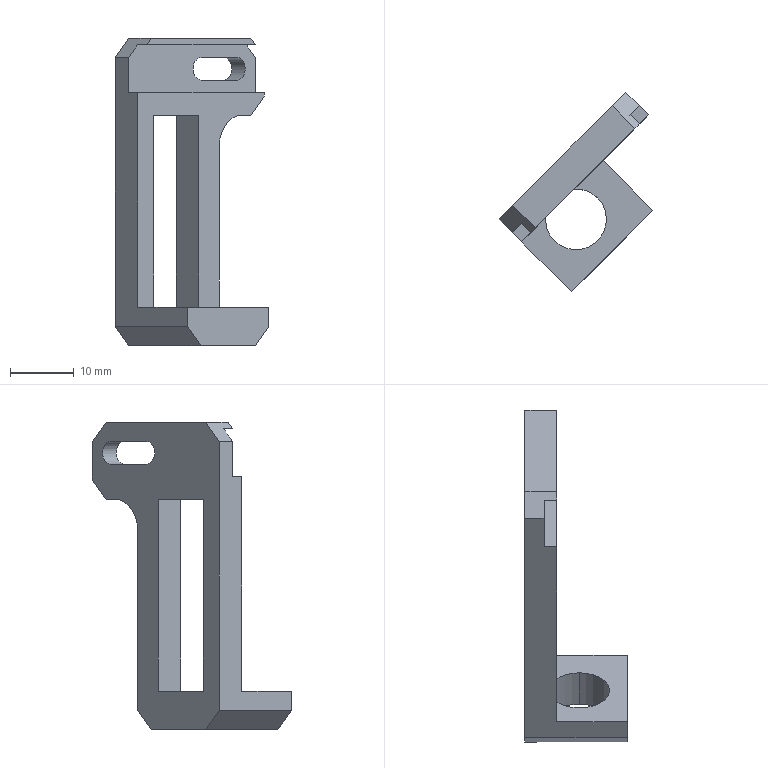Component | SolidWorks | InnerFineAdjustmentBlock-1 | 1 solid | 30 faces | box 24.04 x 31.11 x 48 mm | volume 3473 mm3 | plane 24 | cylinder 6 | commonest cylinder face diameters 3.5 x3 9.5 x2 10 x1
STEP:
#1=COLOUR_RGB('',0.7922,0.8196,0.9333);
#2=FILL_AREA_STYLE_COLOUR('',#1);
#3=FILL_AREA_STYLE('',(#2));
#4=SURFACE_STYLE_FILL_AREA(#3);
#5=SURFACE_SIDE_STYLE('',(#4));
#6=SURFACE_STYLE_USAGE(.BOTH.,#5);
#7=PRESENTATION_STYLE_ASSIGNMENT((#6));
#8=CARTESIAN_POINT('',(-6.312,5.308,0.5823));
#9=VERTEX_POINT('',#8);
#10=CARTESIAN_POINT('',(-6.263,5.357,0.6512));
#11=VERTEX_POINT('',#10);
#12=CARTESIAN_POINT('',(-6.263,5.357,0.5823));
#13=DIRECTION('',(-0.7071,0.7071,0.));
#14=DIRECTION('',(-0.7071,-0.7071,0.));
#15=AXIS2_PLACEMENT_3D('',#12,#13,#14);
#16=CIRCLE('',#15,0.0689);
#17=EDGE_CURVE('',#9,#11,#16,.T.);
#18=ORIENTED_EDGE('',*,*,#17,.F.);
#19=CARTESIAN_POINT('',(-6.395,5.391,0.5823));
#20=VERTEX_POINT('',#19);
#21=CARTESIAN_POINT('',(-5.95,4.946,0.5823));
#22=DIRECTION('',(-0.7071,0.7071,0.));
#23=VECTOR('',#22,39.37);
#24=LINE('',#21,#23);
#25=EDGE_CURVE('',#9,#20,#24,.T.);
#26=ORIENTED_EDGE('',*,*,#25,.T.);
#27=CARTESIAN_POINT('',(-6.347,5.44,0.6512));
#28=VERTEX_POINT('',#27);
#29=CARTESIAN_POINT('',(-6.347,5.44,0.5823));
#30=DIRECTION('',(-0.7071,0.7071,0.));
#31=DIRECTION('',(-0.7071,-0.7071,0.));
#32=AXIS2_PLACEMENT_3D('',#29,#30,#31);
#33=CIRCLE('',#32,0.0689);
#34=EDGE_CURVE('',#20,#28,#33,.T.);
#35=ORIENTED_EDGE('',*,*,#34,.T.);
#36=CARTESIAN_POINT('',(-5.901,4.995,0.6512));
#37=DIRECTION('',(0.7071,-0.7071,-0.));
#38=VECTOR('',#37,39.37);
#39=LINE('',#36,#38);
#40=EDGE_CURVE('',#28,#11,#39,.T.);
#41=ORIENTED_EDGE('',*,*,#40,.T.);
#42=EDGE_LOOP('',(#18,#26,#35,#41));
#43=FACE_OUTER_BOUND('',#42,.T.);
#44=CARTESIAN_POINT('',(-5.901,4.995,0.5823));
#45=DIRECTION('',(-0.7071,0.7071,0.));
#46=DIRECTION('',(-0.7071,-0.7071,0.));
#47=AXIS2_PLACEMENT_3D('',#44,#45,#46);
#48=CYLINDRICAL_SURFACE('',#47,0.0689);
#49=ADVANCED_FACE('',(#43),#48,.F.);
#50=CARTESIAN_POINT('',(-6.451,4.862,-0.8842));
#51=VERTEX_POINT('',#50);
#52=CARTESIAN_POINT('',(-6.187,5.127,-0.8842));
#53=VERTEX_POINT('',#52);
#54=CARTESIAN_POINT('',(-6.319,4.995,-0.8842));
#55=DIRECTION('',(0.,-0.,1.));
#56=DIRECTION('',(-0.7071,-0.7071,0.));
#57=AXIS2_PLACEMENT_3D('',#54,#55,#56);
#58=CIRCLE('',#57,0.187);
#59=EDGE_CURVE('',#51,#53,#58,.T.);
#60=ORIENTED_EDGE('',*,*,#59,.T.);
#61=CARTESIAN_POINT('',(-6.187,5.127,-1.12));
#62=VERTEX_POINT('',#61);
#63=CARTESIAN_POINT('',(-6.187,5.127,-0.7267));
#64=DIRECTION('',(-0.,0.,-1.));
#65=VECTOR('',#64,39.37);
#66=LINE('',#63,#65);
#67=EDGE_CURVE('',#53,#62,#66,.T.);
#68=ORIENTED_EDGE('',*,*,#67,.T.);
#69=CARTESIAN_POINT('',(-6.451,4.862,-1.12));
#70=VERTEX_POINT('',#69);
#71=CARTESIAN_POINT('',(-6.319,4.995,-1.12));
#72=DIRECTION('',(-0.,0.,-1.));
#73=DIRECTION('',(-0.7071,-0.7071,0.));
#74=AXIS2_PLACEMENT_3D('',#71,#72,#73);
#75=CIRCLE('',#74,0.187);
#76=EDGE_CURVE('',#62,#70,#75,.T.);
#77=ORIENTED_EDGE('',*,*,#76,.T.);
#78=CARTESIAN_POINT('',(-6.451,4.862,-0.7267));
#79=DIRECTION('',(-0.,0.,-1.));
#80=VECTOR('',#79,39.37);
#81=LINE('',#78,#80);
#82=EDGE_CURVE('',#51,#70,#81,.T.);
#83=ORIENTED_EDGE('',*,*,#82,.F.);
#84=EDGE_LOOP('',(#60,#68,#77,#83));
#85=FACE_OUTER_BOUND('',#84,.T.);
#86=CARTESIAN_POINT('',(-6.319,4.995,-0.7267));
#87=DIRECTION('',(-0.,0.,-1.));
#88=DIRECTION('',(-0.7071,-0.7071,0.));
#89=AXIS2_PLACEMENT_3D('',#86,#87,#88);
#90=CYLINDRICAL_SURFACE('',#89,0.187);
#91=ADVANCED_FACE('',(#85),#90,.F.);
#92=CARTESIAN_POINT('',(-6.375,5.412,-1.12));
#93=VERTEX_POINT('',#92);
#94=CARTESIAN_POINT('',(-6.291,5.496,-1.002));
#95=VERTEX_POINT('',#94);
#96=CARTESIAN_POINT('',(-6.375,5.412,-1.12));
#97=DIRECTION('',(0.5,0.5,0.7071));
#98=VECTOR('',#97,39.37);
#99=LINE('',#96,#98);
#100=EDGE_CURVE('',#93,#95,#99,.T.);
#101=ORIENTED_EDGE('',*,*,#100,.F.);
#102=CARTESIAN_POINT('',(-6.709,5.078,-1.12));
#103=VERTEX_POINT('',#102);
#104=CARTESIAN_POINT('',(-6.792,4.995,-1.12));
#105=DIRECTION('',(0.7071,0.7071,0.));
#106=VECTOR('',#105,39.37);
#107=LINE('',#104,#106);
#108=EDGE_CURVE('',#103,#93,#107,.T.);
#109=ORIENTED_EDGE('',*,*,#108,.F.);
#110=CARTESIAN_POINT('',(-6.792,4.995,-1.002));
#111=VERTEX_POINT('',#110);
#112=CARTESIAN_POINT('',(-6.792,4.995,-1.002));
#113=DIRECTION('',(0.5,0.5,-0.7071));
#114=VECTOR('',#113,39.37);
#115=LINE('',#112,#114);
#116=EDGE_CURVE('',#111,#103,#115,.T.);
#117=ORIENTED_EDGE('',*,*,#116,.F.);
#118=CARTESIAN_POINT('',(-6.792,4.995,0.6512));
#119=VERTEX_POINT('',#118);
#120=CARTESIAN_POINT('',(-6.792,4.995,-1.12));
#121=DIRECTION('',(-0.,0.,-1.));
#122=VECTOR('',#121,39.37);
#123=LINE('',#120,#122);
#124=EDGE_CURVE('',#119,#111,#123,.T.);
#125=ORIENTED_EDGE('',*,*,#124,.F.);
#126=CARTESIAN_POINT('',(-6.709,5.078,0.7693));
#127=VERTEX_POINT('',#126);
#128=CARTESIAN_POINT('',(-6.709,5.078,0.7693));
#129=DIRECTION('',(-0.5,-0.5,-0.7071));
#130=VECTOR('',#129,39.37);
#131=LINE('',#128,#130);
#132=EDGE_CURVE('',#127,#119,#131,.T.);
#133=ORIENTED_EDGE('',*,*,#132,.F.);
#134=CARTESIAN_POINT('',(-6.096,5.691,0.7693));
#135=VERTEX_POINT('',#134);
#136=CARTESIAN_POINT('',(-6.792,4.995,0.7693));
#137=DIRECTION('',(-0.7071,-0.7071,-0.));
#138=VECTOR('',#137,39.37);
#139=LINE('',#136,#138);
#140=EDGE_CURVE('',#135,#127,#139,.T.);
#141=ORIENTED_EDGE('',*,*,#140,.F.);
#142=CARTESIAN_POINT('',(-6.013,5.774,0.6512));
#143=VERTEX_POINT('',#142);
#144=CARTESIAN_POINT('',(-6.013,5.774,0.6512));
#145=DIRECTION('',(-0.5,-0.5,0.7071));
#146=VECTOR('',#145,39.37);
#147=LINE('',#144,#146);
#148=EDGE_CURVE('',#143,#135,#147,.T.);
#149=ORIENTED_EDGE('',*,*,#148,.F.);
#150=CARTESIAN_POINT('',(-6.013,5.774,0.415));
#151=VERTEX_POINT('',#150);
#152=CARTESIAN_POINT('',(-6.013,5.774,-1.12));
#153=DIRECTION('',(0.,-0.,1.));
#154=VECTOR('',#153,39.37);
#155=LINE('',#152,#154);
#156=EDGE_CURVE('',#151,#143,#155,.T.);
#157=ORIENTED_EDGE('',*,*,#156,.F.);
#158=CARTESIAN_POINT('',(-6.096,5.691,0.2969));
#159=VERTEX_POINT('',#158);
#160=CARTESIAN_POINT('',(-6.096,5.691,0.2969));
#161=DIRECTION('',(0.5,0.5,0.7071));
#162=VECTOR('',#161,39.37);
#163=LINE('',#160,#162);
#164=EDGE_CURVE('',#159,#151,#163,.T.);
#165=ORIENTED_EDGE('',*,*,#164,.F.);
#166=CARTESIAN_POINT('',(-6.152,5.635,0.2969));
#167=VERTEX_POINT('',#166);
#168=CARTESIAN_POINT('',(-6.792,4.995,0.2969));
#169=DIRECTION('',(0.7071,0.7071,0.));
#170=VECTOR('',#169,39.37);
#171=LINE('',#168,#170);
#172=EDGE_CURVE('',#167,#159,#171,.T.);
#173=ORIENTED_EDGE('',*,*,#172,.F.);
#174=CARTESIAN_POINT('',(-6.291,5.496,0.1));
#175=VERTEX_POINT('',#174);
#176=CARTESIAN_POINT('',(-6.152,5.635,0.1));
#177=DIRECTION('',(-0.7071,0.7071,0.));
#178=DIRECTION('',(0.7071,0.7071,0.));
#179=AXIS2_PLACEMENT_3D('',#176,#177,#178);
#180=CIRCLE('',#179,0.1969);
#181=EDGE_CURVE('',#175,#167,#180,.T.);
#182=ORIENTED_EDGE('',*,*,#181,.F.);
#183=CARTESIAN_POINT('',(-6.291,5.496,-1.12));
#184=DIRECTION('',(0.,-0.,1.));
#185=VECTOR('',#184,39.37);
#186=LINE('',#183,#185);
#187=EDGE_CURVE('',#95,#175,#186,.T.);
#188=ORIENTED_EDGE('',*,*,#187,.F.);
#189=EDGE_LOOP('',(#101,#109,#117,#125,#133,#141,#149,#157,#165,#173,#182,#188));
#190=FACE_OUTER_BOUND('',#189,.T.);
#191=CARTESIAN_POINT('',(-6.416,5.371,-0.8842));
#192=VERTEX_POINT('',#191);
#193=CARTESIAN_POINT('',(-6.695,5.092,-0.8842));
#194=VERTEX_POINT('',#193);
#195=CARTESIAN_POINT('',(-6.792,4.995,-0.8842));
#196=DIRECTION('',(-0.7071,-0.7071,-0.));
#197=VECTOR('',#196,39.37);
#198=LINE('',#195,#197);
#199=EDGE_CURVE('',#192,#194,#198,.T.);
#200=ORIENTED_EDGE('',*,*,#199,.F.);
#201=CARTESIAN_POINT('',(-6.416,5.371,0.2969));
#202=VERTEX_POINT('',#201);
#203=CARTESIAN_POINT('',(-6.416,5.371,-1.12));
#204=DIRECTION('',(-0.,0.,-1.));
#205=VECTOR('',#204,39.37);
#206=LINE('',#203,#205);
#207=EDGE_CURVE('',#202,#192,#206,.T.);
#208=ORIENTED_EDGE('',*,*,#207,.F.);
#209=CARTESIAN_POINT('',(-6.695,5.092,0.2969));
#210=VERTEX_POINT('',#209);
#211=CARTESIAN_POINT('',(-6.792,4.995,0.2969));
#212=DIRECTION('',(0.7071,0.7071,0.));
#213=VECTOR('',#212,39.37);
#214=LINE('',#211,#213);
#215=EDGE_CURVE('',#210,#202,#214,.T.);
#216=ORIENTED_EDGE('',*,*,#215,.F.);
#217=CARTESIAN_POINT('',(-6.695,5.092,-1.12));
#218=DIRECTION('',(0.,-0.,1.));
#219=VECTOR('',#218,39.37);
#220=LINE('',#217,#219);
#221=EDGE_CURVE('',#194,#210,#220,.T.);
#222=ORIENTED_EDGE('',*,*,#221,.F.);
#223=EDGE_LOOP('',(#200,#208,#216,#222));
#224=FACE_BOUND('',#223,.T.);
#225=CARTESIAN_POINT('',(-6.124,5.663,0.6512));
#226=VERTEX_POINT('',#225);
#227=CARTESIAN_POINT('',(-6.124,5.663,0.5134));
#228=VERTEX_POINT('',#227);
#229=CARTESIAN_POINT('',(-6.124,5.663,0.5823));
#230=DIRECTION('',(-0.7071,0.7071,0.));
#231=DIRECTION('',(-0.7071,-0.7071,0.));
#232=AXIS2_PLACEMENT_3D('',#229,#230,#231);
#233=CIRCLE('',#232,0.0689);
#234=EDGE_CURVE('',#226,#228,#233,.T.);
#235=ORIENTED_EDGE('',*,*,#234,.F.);
#236=CARTESIAN_POINT('',(-6.792,4.995,0.6512));
#237=DIRECTION('',(0.7071,0.7071,0.));
#238=VECTOR('',#237,39.37);
#239=LINE('',#236,#238);
#240=EDGE_CURVE('',#28,#226,#239,.T.);
#241=ORIENTED_EDGE('',*,*,#240,.F.);
#242=ORIENTED_EDGE('',*,*,#34,.F.);
#243=CARTESIAN_POINT('',(-6.347,5.44,0.5134));
#244=VERTEX_POINT('',#243);
#245=CARTESIAN_POINT('',(-6.347,5.44,0.5823));
#246=DIRECTION('',(-0.7071,0.7071,0.));
#247=DIRECTION('',(-0.7071,-0.7071,0.));
#248=AXIS2_PLACEMENT_3D('',#245,#246,#247);
#249=CIRCLE('',#248,0.0689);
#250=EDGE_CURVE('',#244,#20,#249,.T.);
#251=ORIENTED_EDGE('',*,*,#250,.F.);
#252=CARTESIAN_POINT('',(-6.792,4.995,0.5134));
#253=DIRECTION('',(-0.7071,-0.7071,-0.));
#254=VECTOR('',#253,39.37);
#255=LINE('',#252,#254);
#256=EDGE_CURVE('',#228,#244,#255,.T.);
#257=ORIENTED_EDGE('',*,*,#256,.F.);
#258=EDGE_LOOP('',(#235,#241,#242,#251,#257));
#259=FACE_BOUND('',#258,.T.);
#260=CARTESIAN_POINT('',(-6.792,4.995,-1.12));
#261=DIRECTION('',(0.7071,-0.7071,-0.));
#262=DIRECTION('',(0.7071,0.7071,0.));
#263=AXIS2_PLACEMENT_3D('',#260,#261,#262);
#264=PLANE('',#263);
#265=ADVANCED_FACE('',(#190,#224,#259),#264,.F.);
#266=CARTESIAN_POINT('',(-5.846,5.05,-1.002));
#267=VERTEX_POINT('',#266);
#268=CARTESIAN_POINT('',(-5.846,5.05,-1.002));
#269=DIRECTION('',(0.7071,-0.7071,-0.));
#270=VECTOR('',#269,39.37);
#271=LINE('',#268,#270);
#272=EDGE_CURVE('',#95,#267,#271,.T.);
#273=ORIENTED_EDGE('',*,*,#272,.F.);
#274=ORIENTED_EDGE('',*,*,#187,.T.);
#275=CARTESIAN_POINT('',(-6.152,5.357,0.1));
#276=VERTEX_POINT('',#275);
#277=CARTESIAN_POINT('',(-5.846,5.05,0.1));
#278=DIRECTION('',(-0.7071,0.7071,0.));
#279=VECTOR('',#278,39.37);
#280=LINE('',#277,#279);
#281=EDGE_CURVE('',#276,#175,#280,.T.);
#282=ORIENTED_EDGE('',*,*,#281,.F.);
#283=CARTESIAN_POINT('',(-6.152,5.357,-0.8842));
#284=VERTEX_POINT('',#283);
#285=CARTESIAN_POINT('',(-6.152,5.357,-1.12));
#286=DIRECTION('',(0.,-0.,1.));
#287=VECTOR('',#286,39.37);
#288=LINE('',#285,#287);
#289=EDGE_CURVE('',#284,#276,#288,.T.);
#290=ORIENTED_EDGE('',*,*,#289,.F.);
#291=CARTESIAN_POINT('',(-5.846,5.05,-0.8842));
#292=VERTEX_POINT('',#291);
#293=CARTESIAN_POINT('',(-5.846,5.05,-0.8842));
#294=DIRECTION('',(-0.7071,0.7071,0.));
#295=VECTOR('',#294,39.37);
#296=LINE('',#293,#295);
#297=EDGE_CURVE('',#292,#284,#296,.T.);
#298=ORIENTED_EDGE('',*,*,#297,.F.);
#299=CARTESIAN_POINT('',(-5.846,5.05,-1.12));
#300=DIRECTION('',(0.,-0.,1.));
#301=VECTOR('',#300,39.37);
#302=LINE('',#299,#301);
#303=EDGE_CURVE('',#267,#292,#302,.T.);
#304=ORIENTED_EDGE('',*,*,#303,.F.);
#305=EDGE_LOOP('',(#273,#274,#282,#290,#298,#304));
#306=FACE_OUTER_BOUND('',#305,.T.);
#307=CARTESIAN_POINT('',(-5.846,5.05,-1.12));
#308=DIRECTION('',(-0.7071,-0.7071,-0.));
#309=DIRECTION('',(0.,-0.,1.));
#310=AXIS2_PLACEMENT_3D('',#307,#308,#309);
#311=PLANE('',#310);
#312=ADVANCED_FACE('',(#306),#311,.F.);
#313=CARTESIAN_POINT('',(-5.929,4.967,-1.12));
#314=VERTEX_POINT('',#313);
#315=CARTESIAN_POINT('',(-5.929,4.967,-1.12));
#316=DIRECTION('',(0.7071,-0.7071,-0.));
#317=VECTOR('',#316,39.37);
#318=LINE('',#315,#317);
#319=EDGE_CURVE('',#93,#314,#318,.T.);
#320=ORIENTED_EDGE('',*,*,#319,.F.);
#321=ORIENTED_EDGE('',*,*,#100,.T.);
#322=ORIENTED_EDGE('',*,*,#272,.T.);
#323=CARTESIAN_POINT('',(-5.846,5.05,-1.002));
#324=DIRECTION('',(0.5,0.5,0.7071));
#325=VECTOR('',#324,39.37);
#326=LINE('',#323,#325);
#327=EDGE_CURVE('',#314,#267,#326,.T.);
#328=ORIENTED_EDGE('',*,*,#327,.F.);
#329=EDGE_LOOP('',(#320,#321,#322,#328));
#330=FACE_OUTER_BOUND('',#329,.T.);
#331=CARTESIAN_POINT('',(-5.846,5.05,-1.002));
#332=DIRECTION('',(-0.5,-0.5,0.7071));
#333=DIRECTION('',(0.5,0.5,0.7071));
#334=AXIS2_PLACEMENT_3D('',#331,#332,#333);
#335=PLANE('',#334);
#336=ADVANCED_FACE('',(#330),#335,.F.);
#337=ORIENTED_EDGE('',*,*,#319,.T.);
#338=CARTESIAN_POINT('',(-6.263,4.633,-1.12));
#339=VERTEX_POINT('',#338);
#340=CARTESIAN_POINT('',(-6.347,4.549,-1.12));
#341=DIRECTION('',(0.7071,0.7071,0.));
#342=VECTOR('',#341,39.37);
#343=LINE('',#340,#342);
#344=EDGE_CURVE('',#339,#314,#343,.T.);
#345=ORIENTED_EDGE('',*,*,#344,.F.);
#346=CARTESIAN_POINT('',(-6.709,5.078,-1.12));
#347=DIRECTION('',(0.7071,-0.7071,-0.));
#348=VECTOR('',#347,39.37);
#349=LINE('',#346,#348);
#350=EDGE_CURVE('',#103,#339,#349,.T.);
#351=ORIENTED_EDGE('',*,*,#350,.F.);
#352=ORIENTED_EDGE('',*,*,#108,.T.);
#353=EDGE_LOOP('',(#337,#345,#351,#352));
#354=FACE_OUTER_BOUND('',#353,.T.);
#355=CARTESIAN_POINT('',(-6.319,4.995,-1.12));
#356=DIRECTION('',(-0.,0.,-1.));
#357=DIRECTION('',(-0.7071,-0.7071,0.));
#358=AXIS2_PLACEMENT_3D('',#355,#356,#357);
#359=CIRCLE('',#358,0.187);
#360=EDGE_CURVE('',#70,#62,#359,.T.);
#361=ORIENTED_EDGE('',*,*,#360,.F.);
#362=ORIENTED_EDGE('',*,*,#76,.F.);
#363=EDGE_LOOP('',(#361,#362));
#364=FACE_BOUND('',#363,.T.);
#365=CARTESIAN_POINT('',(-6.792,4.995,-1.12));
#366=DIRECTION('',(0.,-0.,1.));
#367=DIRECTION('',(0.7071,0.7071,0.));
#368=AXIS2_PLACEMENT_3D('',#365,#366,#367);
#369=PLANE('',#368);
#370=ADVANCED_FACE('',(#354,#364),#369,.F.);
#371=ORIENTED_EDGE('',*,*,#350,.T.);
#372=CARTESIAN_POINT('',(-6.347,4.549,-1.002));
#373=VERTEX_POINT('',#372);
#374=CARTESIAN_POINT('',(-6.347,4.549,-1.002));
#375=DIRECTION('',(0.5,0.5,-0.7071));
#376=VECTOR('',#375,39.37);
#377=LINE('',#374,#376);
#378=EDGE_CURVE('',#373,#339,#377,.T.);
#379=ORIENTED_EDGE('',*,*,#378,.F.);
#380=CARTESIAN_POINT('',(-6.792,4.995,-1.002));
#381=DIRECTION('',(0.7071,-0.7071,-0.));
#382=VECTOR('',#381,39.37);
#383=LINE('',#380,#382);
#384=EDGE_CURVE('',#111,#373,#383,.T.);
#385=ORIENTED_EDGE('',*,*,#384,.F.);
#386=ORIENTED_EDGE('',*,*,#116,.T.);
#387=EDGE_LOOP('',(#371,#379,#385,#386));
#388=FACE_OUTER_BOUND('',#387,.T.);
#389=CARTESIAN_POINT('',(-6.792,4.995,-1.002));
#390=DIRECTION('',(0.5,0.5,0.7071));
#391=DIRECTION('',(0.5,0.5,-0.7071));
#392=AXIS2_PLACEMENT_3D('',#389,#390,#391);
#393=PLANE('',#392);
#394=ADVANCED_FACE('',(#388),#393,.F.);
#395=CARTESIAN_POINT('',(-6.709,4.911,0.6512));
#396=VERTEX_POINT('',#395);
#397=CARTESIAN_POINT('',(-6.792,4.995,0.6512));
#398=DIRECTION('',(0.7071,-0.7071,-0.));
#399=VECTOR('',#398,39.37);
#400=LINE('',#397,#399);
#401=EDGE_CURVE('',#119,#396,#400,.T.);
#402=ORIENTED_EDGE('',*,*,#401,.F.);
#403=ORIENTED_EDGE('',*,*,#124,.T.);
#404=ORIENTED_EDGE('',*,*,#384,.T.);
#405=CARTESIAN_POINT('',(-6.347,4.549,-0.8842));
#406=VERTEX_POINT('',#405);
#407=CARTESIAN_POINT('',(-6.347,4.549,-1.12));
#408=DIRECTION('',(-0.,0.,-1.));
#409=VECTOR('',#408,39.37);
#410=LINE('',#407,#409);
#411=EDGE_CURVE('',#406,#373,#410,.T.);
#412=ORIENTED_EDGE('',*,*,#411,.F.);
#413=CARTESIAN_POINT('',(-6.653,4.856,-0.8842));
#414=VERTEX_POINT('',#413);
#415=CARTESIAN_POINT('',(-6.792,4.995,-0.8842));
#416=DIRECTION('',(0.7071,-0.7071,-0.));
#417=VECTOR('',#416,39.37);
#418=LINE('',#415,#417);
#419=EDGE_CURVE('',#414,#406,#418,.T.);
#420=ORIENTED_EDGE('',*,*,#419,.F.);
#421=CARTESIAN_POINT('',(-6.653,4.856,0.4347));
#422=VERTEX_POINT('',#421);
#423=CARTESIAN_POINT('',(-6.653,4.856,-1.12));
#424=DIRECTION('',(-0.,0.,-1.));
#425=VECTOR('',#424,39.37);
#426=LINE('',#423,#425);
#427=EDGE_CURVE('',#422,#414,#426,.T.);
#428=ORIENTED_EDGE('',*,*,#427,.F.);
#429=CARTESIAN_POINT('',(-6.709,4.911,0.4347));
#430=VERTEX_POINT('',#429);
#431=CARTESIAN_POINT('',(-6.792,4.995,0.4347));
#432=DIRECTION('',(0.7071,-0.7071,-0.));
#433=VECTOR('',#432,39.37);
#434=LINE('',#431,#433);
#435=EDGE_CURVE('',#430,#422,#434,.T.);
#436=ORIENTED_EDGE('',*,*,#435,.F.);
#437=CARTESIAN_POINT('',(-6.709,4.911,-1.12));
#438=DIRECTION('',(-0.,0.,-1.));
#439=VECTOR('',#438,39.37);
#440=LINE('',#437,#439);
#441=EDGE_CURVE('',#396,#430,#440,.T.);
#442=ORIENTED_EDGE('',*,*,#441,.F.);
#443=EDGE_LOOP('',(#402,#403,#404,#412,#420,#428,#436,#442));
#444=FACE_OUTER_BOUND('',#443,.T.);
#445=CARTESIAN_POINT('',(-6.792,4.995,-1.12));
#446=DIRECTION('',(0.7071,0.7071,0.));
#447=DIRECTION('',(-0.,0.,-1.));
#448=AXIS2_PLACEMENT_3D('',#445,#446,#447);
#449=PLANE('',#448);
#450=ADVANCED_FACE('',(#444),#449,.F.);
#451=ORIENTED_EDGE('',*,*,#401,.T.);
#452=CARTESIAN_POINT('',(-6.653,4.967,0.73));
#453=VERTEX_POINT('',#452);
#454=CARTESIAN_POINT('',(-6.625,4.995,0.7693));
#455=DIRECTION('',(-0.5,-0.5,-0.7071));
#456=VECTOR('',#455,39.37);
#457=LINE('',#454,#456);
#458=EDGE_CURVE('',#453,#396,#457,.T.);
#459=ORIENTED_EDGE('',*,*,#458,.F.);
#460=CARTESIAN_POINT('',(-6.597,4.911,0.73));
#461=VERTEX_POINT('',#460);
#462=CARTESIAN_POINT('',(-6.736,5.05,0.73));
#463=DIRECTION('',(-0.7071,0.7071,0.));
#464=VECTOR('',#463,39.37);
#465=LINE('',#462,#464);
#466=EDGE_CURVE('',#461,#453,#465,.T.);
#467=ORIENTED_EDGE('',*,*,#466,.F.);
#468=CARTESIAN_POINT('',(-6.569,4.939,0.7693));
#469=VERTEX_POINT('',#468);
#470=CARTESIAN_POINT('',(-6.569,4.939,0.7693));
#471=DIRECTION('',(-0.5,-0.5,-0.7071));
#472=VECTOR('',#471,39.37);
#473=LINE('',#470,#472);
#474=EDGE_CURVE('',#469,#461,#473,.T.);
#475=ORIENTED_EDGE('',*,*,#474,.F.);
#476=CARTESIAN_POINT('',(-6.709,5.078,0.7693));
#477=DIRECTION('',(0.7071,-0.7071,-0.));
#478=VECTOR('',#477,39.37);
#479=LINE('',#476,#478);
#480=EDGE_CURVE('',#127,#469,#479,.T.);
#481=ORIENTED_EDGE('',*,*,#480,.F.);
#482=ORIENTED_EDGE('',*,*,#132,.T.);
#483=EDGE_LOOP('',(#451,#459,#467,#475,#481,#482));
#484=FACE_OUTER_BOUND('',#483,.T.);
#485=CARTESIAN_POINT('',(-6.709,5.078,0.7693));
#486=DIRECTION('',(0.5,0.5,-0.7071));
#487=DIRECTION('',(-0.5,-0.5,-0.7071));
#488=AXIS2_PLACEMENT_3D('',#485,#486,#487);
#489=PLANE('',#488);
#490=ADVANCED_FACE('',(#484),#489,.F.);
#491=CARTESIAN_POINT('',(-5.957,5.551,0.7693));
#492=VERTEX_POINT('',#491);
#493=CARTESIAN_POINT('',(-6.096,5.691,0.7693));
#494=DIRECTION('',(0.7071,-0.7071,-0.));
#495=VECTOR('',#494,39.37);
#496=LINE('',#493,#495);
#497=EDGE_CURVE('',#135,#492,#496,.T.);
#498=ORIENTED_EDGE('',*,*,#497,.F.);
#499=ORIENTED_EDGE('',*,*,#140,.T.);
#500=ORIENTED_EDGE('',*,*,#480,.T.);
#501=CARTESIAN_POINT('',(-6.653,4.856,0.7693));
#502=DIRECTION('',(-0.7071,-0.7071,-0.));
#503=VECTOR('',#502,39.37);
#504=LINE('',#501,#503);
#505=EDGE_CURVE('',#492,#469,#504,.T.);
#506=ORIENTED_EDGE('',*,*,#505,.F.);
#507=EDGE_LOOP('',(#498,#499,#500,#506));
#508=FACE_OUTER_BOUND('',#507,.T.);
#509=CARTESIAN_POINT('',(-6.792,4.995,0.7693));
#510=DIRECTION('',(-0.,0.,-1.));
#511=DIRECTION('',(-0.7071,-0.7071,-0.));
#512=AXIS2_PLACEMENT_3D('',#509,#510,#511);
#513=PLANE('',#512);
#514=ADVANCED_FACE('',(#508),#513,.F.);
#515=ORIENTED_EDGE('',*,*,#497,.T.);
#516=CARTESIAN_POINT('',(-5.929,5.579,0.73));
#517=VERTEX_POINT('',#516);
#518=CARTESIAN_POINT('',(-5.873,5.635,0.6512));
#519=DIRECTION('',(-0.5,-0.5,0.7071));
#520=VECTOR('',#519,39.37);
#521=LINE('',#518,#520);
#522=EDGE_CURVE('',#517,#492,#521,.T.);
#523=ORIENTED_EDGE('',*,*,#522,.F.);
#524=CARTESIAN_POINT('',(-5.985,5.635,0.73));
#525=VERTEX_POINT('',#524);
#526=CARTESIAN_POINT('',(-6.068,5.719,0.73));
#527=DIRECTION('',(0.7071,-0.7071,-0.));
#528=VECTOR('',#527,39.37);
#529=LINE('',#526,#528);
#530=EDGE_CURVE('',#525,#517,#529,.T.);
#531=ORIENTED_EDGE('',*,*,#530,.F.);
#532=CARTESIAN_POINT('',(-5.929,5.691,0.6512));
#533=VERTEX_POINT('',#532);
#534=CARTESIAN_POINT('',(-5.929,5.691,0.6512));
#535=DIRECTION('',(-0.5,-0.5,0.7071));
#536=VECTOR('',#535,39.37);
#537=LINE('',#534,#536);
#538=EDGE_CURVE('',#533,#525,#537,.T.);
#539=ORIENTED_EDGE('',*,*,#538,.F.);
#540=CARTESIAN_POINT('',(-6.013,5.774,0.6512));
#541=DIRECTION('',(0.7071,-0.7071,-0.));
#542=VECTOR('',#541,39.37);
#543=LINE('',#540,#542);
#544=EDGE_CURVE('',#143,#533,#543,.T.);
#545=ORIENTED_EDGE('',*,*,#544,.F.);
#546=ORIENTED_EDGE('',*,*,#148,.T.);
#547=EDGE_LOOP('',(#515,#523,#531,#539,#545,#546));
#548=FACE_OUTER_BOUND('',#547,.T.);
#549=CARTESIAN_POINT('',(-6.013,5.774,0.6512));
#550=DIRECTION('',(-0.5,-0.5,-0.7071));
#551=DIRECTION('',(-0.5,-0.5,0.7071));
#552=AXIS2_PLACEMENT_3D('',#549,#550,#551);
#553=PLANE('',#552);
#554=ADVANCED_FACE('',(#548),#553,.F.);
#555=CARTESIAN_POINT('',(-5.873,5.635,0.415));
#556=VERTEX_POINT('',#555);
#557=CARTESIAN_POINT('',(-6.013,5.774,0.415));
#558=DIRECTION('',(0.7071,-0.7071,-0.));
#559=VECTOR('',#558,39.37);
#560=LINE('',#557,#559);
#561=EDGE_CURVE('',#151,#556,#560,.T.);
#562=ORIENTED_EDGE('',*,*,#561,.F.);
#563=ORIENTED_EDGE('',*,*,#156,.T.);
#564=ORIENTED_EDGE('',*,*,#544,.T.);
#565=CARTESIAN_POINT('',(-5.929,5.691,0.4347));
#566=VERTEX_POINT('',#565);
#567=CARTESIAN_POINT('',(-5.929,5.691,-1.12));
#568=DIRECTION('',(0.,-0.,1.));
#569=VECTOR('',#568,39.37);
#570=LINE('',#567,#569);
#571=EDGE_CURVE('',#566,#533,#570,.T.);
#572=ORIENTED_EDGE('',*,*,#571,.F.);
#573=CARTESIAN_POINT('',(-5.873,5.635,0.4347));
#574=VERTEX_POINT('',#573);
#575=CARTESIAN_POINT('',(-6.013,5.774,0.4347));
#576=DIRECTION('',(-0.7071,0.7071,0.));
#577=VECTOR('',#576,39.37);
#578=LINE('',#575,#577);
#579=EDGE_CURVE('',#574,#566,#578,.T.);
#580=ORIENTED_EDGE('',*,*,#579,.F.);
#581=CARTESIAN_POINT('',(-5.873,5.635,-1.12));
#582=DIRECTION('',(0.,-0.,1.));
#583=VECTOR('',#582,39.37);
#584=LINE('',#581,#583);
#585=EDGE_CURVE('',#556,#574,#584,.T.);
#586=ORIENTED_EDGE('',*,*,#585,.F.);
#587=EDGE_LOOP('',(#562,#563,#564,#572,#580,#586));
#588=FACE_OUTER_BOUND('',#587,.T.);
#589=CARTESIAN_POINT('',(-6.013,5.774,-1.12));
#590=DIRECTION('',(-0.7071,-0.7071,-0.));
#591=DIRECTION('',(0.,-0.,1.));
#592=AXIS2_PLACEMENT_3D('',#589,#590,#591);
#593=PLANE('',#592);
#594=ADVANCED_FACE('',(#588),#593,.F.);
#595=CARTESIAN_POINT('',(-5.957,5.551,0.2969));
#596=VERTEX_POINT('',#595);
#597=CARTESIAN_POINT('',(-6.096,5.691,0.2969));
#598=DIRECTION('',(0.7071,-0.7071,-0.));
#599=VECTOR('',#598,39.37);
#600=LINE('',#597,#599);
#601=EDGE_CURVE('',#159,#596,#600,.T.);
#602=ORIENTED_EDGE('',*,*,#601,.F.);
#603=ORIENTED_EDGE('',*,*,#164,.T.);
#604=ORIENTED_EDGE('',*,*,#561,.T.);
#605=CARTESIAN_POINT('',(-5.873,5.635,0.415));
#606=DIRECTION('',(0.5,0.5,0.7071));
#607=VECTOR('',#606,39.37);
#608=LINE('',#605,#607);
#609=EDGE_CURVE('',#596,#556,#608,.T.);
#610=ORIENTED_EDGE('',*,*,#609,.F.);
#611=EDGE_LOOP('',(#602,#603,#604,#610));
#612=FACE_OUTER_BOUND('',#611,.T.);
#613=CARTESIAN_POINT('',(-6.013,5.774,0.415));
#614=DIRECTION('',(-0.5,-0.5,0.7071));
#615=DIRECTION('',(0.5,0.5,0.7071));
#616=AXIS2_PLACEMENT_3D('',#613,#614,#615);
#617=PLANE('',#616);
#618=ADVANCED_FACE('',(#612),#617,.F.);
#619=ORIENTED_EDGE('',*,*,#601,.T.);
#620=CARTESIAN_POINT('',(-6.013,5.496,0.2969));
#621=VERTEX_POINT('',#620);
#622=CARTESIAN_POINT('',(-5.873,5.635,0.2969));
#623=DIRECTION('',(0.7071,0.7071,0.));
#624=VECTOR('',#623,39.37);
#625=LINE('',#622,#624);
#626=EDGE_CURVE('',#621,#596,#625,.T.);
#627=ORIENTED_EDGE('',*,*,#626,.F.);
#628=CARTESIAN_POINT('',(-5.873,5.357,0.2969));
#629=DIRECTION('',(0.7071,-0.7071,-0.));
#630=VECTOR('',#629,39.37);
#631=LINE('',#628,#630);
#632=EDGE_CURVE('',#167,#621,#631,.T.);
#633=ORIENTED_EDGE('',*,*,#632,.F.);
#634=ORIENTED_EDGE('',*,*,#172,.T.);
#635=EDGE_LOOP('',(#619,#627,#633,#634));
#636=FACE_OUTER_BOUND('',#635,.T.);
#637=CARTESIAN_POINT('',(-5.734,5.496,0.2969));
#638=DIRECTION('',(0.,-0.,1.));
#639=DIRECTION('',(0.7071,0.7071,0.));
#640=AXIS2_PLACEMENT_3D('',#637,#638,#639);
#641=PLANE('',#640);
#642=ADVANCED_FACE('',(#636),#641,.F.);
#643=ORIENTED_EDGE('',*,*,#281,.T.);
#644=ORIENTED_EDGE('',*,*,#181,.T.);
#645=ORIENTED_EDGE('',*,*,#632,.T.);
#646=CARTESIAN_POINT('',(-6.013,5.496,0.1));
#647=DIRECTION('',(-0.7071,0.7071,0.));
#648=DIRECTION('',(0.7071,0.7071,0.));
#649=AXIS2_PLACEMENT_3D('',#646,#647,#648);
#650=CIRCLE('',#649,0.1969);
#651=EDGE_CURVE('',#276,#621,#650,.T.);
#652=ORIENTED_EDGE('',*,*,#651,.F.);
#653=EDGE_LOOP('',(#643,#644,#645,#652));
#654=FACE_OUTER_BOUND('',#653,.T.);
#655=CARTESIAN_POINT('',(-5.873,5.357,0.1));
#656=DIRECTION('',(0.7071,-0.7071,-0.));
#657=DIRECTION('',(0.7071,0.7071,0.));
#658=AXIS2_PLACEMENT_3D('',#655,#656,#657);
#659=CYLINDRICAL_SURFACE('',#658,0.1969);
#660=ADVANCED_FACE('',(#654),#659,.F.);
#661=CARTESIAN_POINT('',(-6.555,4.953,-0.8842));
#662=VERTEX_POINT('',#661);
#663=CARTESIAN_POINT('',(-6.249,4.647,-0.8842));
#664=DIRECTION('',(0.7071,-0.7071,-0.));
#665=VECTOR('',#664,39.37);
#666=LINE('',#663,#665);
#667=EDGE_CURVE('',#194,#662,#666,.T.);
#668=ORIENTED_EDGE('',*,*,#667,.F.);
#669=ORIENTED_EDGE('',*,*,#221,.T.);
#670=CARTESIAN_POINT('',(-6.555,4.953,0.2969));
#671=VERTEX_POINT('',#670);
#672=CARTESIAN_POINT('',(-6.249,4.647,0.2969));
#673=DIRECTION('',(-0.7071,0.7071,0.));
#674=VECTOR('',#673,39.37);
#675=LINE('',#672,#674);
#676=EDGE_CURVE('',#671,#210,#675,.T.);
#677=ORIENTED_EDGE('',*,*,#676,.F.);
#678=CARTESIAN_POINT('',(-6.555,4.953,-0.8842));
#679=DIRECTION('',(0.,-0.,1.));
#680=VECTOR('',#679,39.37);
#681=LINE('',#678,#680);
#682=EDGE_CURVE('',#662,#671,#681,.T.);
#683=ORIENTED_EDGE('',*,*,#682,.F.);
#684=EDGE_LOOP('',(#668,#669,#677,#683));
#685=FACE_OUTER_BOUND('',#684,.T.);
#686=CARTESIAN_POINT('',(-6.249,4.647,-0.8842));
#687=DIRECTION('',(-0.7071,-0.7071,-0.));
#688=DIRECTION('',(0.,-0.,1.));
#689=AXIS2_PLACEMENT_3D('',#686,#687,#688);
#690=PLANE('',#689);
#691=ADVANCED_FACE('',(#685),#690,.F.);
#692=CARTESIAN_POINT('',(-6.347,4.549,-0.8842));
#693=DIRECTION('',(-0.7071,-0.7071,-0.));
#694=VECTOR('',#693,39.37);
#695=LINE('',#692,#694);
#696=EDGE_CURVE('',#292,#406,#695,.T.);
#697=ORIENTED_EDGE('',*,*,#696,.F.);
#698=ORIENTED_EDGE('',*,*,#297,.T.);
#699=CARTESIAN_POINT('',(-6.277,5.231,-0.8842));
#700=VERTEX_POINT('',#699);
#701=CARTESIAN_POINT('',(-6.653,4.856,-0.8842));
#702=DIRECTION('',(0.7071,0.7071,0.));
#703=VECTOR('',#702,39.37);
#704=LINE('',#701,#703);
#705=EDGE_CURVE('',#700,#284,#704,.T.);
#706=ORIENTED_EDGE('',*,*,#705,.F.);
#707=CARTESIAN_POINT('',(-5.971,4.925,-0.8842));
#708=DIRECTION('',(0.7071,-0.7071,-0.));
#709=VECTOR('',#708,39.37);
#710=LINE('',#707,#709);
#711=EDGE_CURVE('',#192,#700,#710,.T.);
#712=ORIENTED_EDGE('',*,*,#711,.F.);
#713=ORIENTED_EDGE('',*,*,#199,.T.);
#714=ORIENTED_EDGE('',*,*,#667,.T.);
#715=CARTESIAN_POINT('',(-6.653,4.856,-0.8842));
#716=DIRECTION('',(0.7071,0.7071,0.));
#717=VECTOR('',#716,39.37);
#718=LINE('',#715,#717);
#719=EDGE_CURVE('',#414,#662,#718,.T.);
#720=ORIENTED_EDGE('',*,*,#719,.F.);
#721=ORIENTED_EDGE('',*,*,#419,.T.);
#722=EDGE_LOOP('',(#697,#698,#706,#712,#713,#714,#720,#721));
#723=FACE_OUTER_BOUND('',#722,.T.);
#724=ORIENTED_EDGE('',*,*,#59,.F.);
#725=CARTESIAN_POINT('',(-6.319,4.995,-0.8842));
#726=DIRECTION('',(0.,-0.,1.));
#727=DIRECTION('',(-0.7071,-0.7071,0.));
#728=AXIS2_PLACEMENT_3D('',#725,#726,#727);
#729=CIRCLE('',#728,0.187);
#730=EDGE_CURVE('',#53,#51,#729,.T.);
#731=ORIENTED_EDGE('',*,*,#730,.F.);
#732=EDGE_LOOP('',(#724,#731));
#733=FACE_BOUND('',#732,.T.);
#734=CARTESIAN_POINT('',(-6.347,4.549,-0.8842));
#735=DIRECTION('',(0.,0.,-1.));
#736=DIRECTION('',(-0.7071,-0.7071,-0.));
#737=AXIS2_PLACEMENT_3D('',#734,#735,#736);
#738=PLANE('',#737);
#739=ADVANCED_FACE('',(#723,#733),#738,.F.);
#740=CARTESIAN_POINT('',(-6.277,5.231,0.2969));
#741=VERTEX_POINT('',#740);
#742=CARTESIAN_POINT('',(-5.971,4.925,0.2969));
#743=DIRECTION('',(0.7071,-0.7071,-0.));
#744=VECTOR('',#743,39.37);
#745=LINE('',#742,#744);
#746=EDGE_CURVE('',#202,#741,#745,.T.);
#747=ORIENTED_EDGE('',*,*,#746,.F.);
#748=ORIENTED_EDGE('',*,*,#207,.T.);
#749=ORIENTED_EDGE('',*,*,#711,.T.);
#750=CARTESIAN_POINT('',(-6.277,5.231,-0.8842));
#751=DIRECTION('',(-0.,0.,-1.));
#752=VECTOR('',#751,39.37);
#753=LINE('',#750,#752);
#754=EDGE_CURVE('',#741,#700,#753,.T.);
#755=ORIENTED_EDGE('',*,*,#754,.F.);
#756=EDGE_LOOP('',(#747,#748,#749,#755));
#757=FACE_OUTER_BOUND('',#756,.T.);
#758=CARTESIAN_POINT('',(-5.971,4.925,-0.8842));
#759=DIRECTION('',(0.7071,0.7071,0.));
#760=DIRECTION('',(-0.,0.,-1.));
#761=AXIS2_PLACEMENT_3D('',#758,#759,#760);
#762=PLANE('',#761);
#763=ADVANCED_FACE('',(#757),#762,.F.);
#764=ORIENTED_EDGE('',*,*,#676,.T.);
#765=ORIENTED_EDGE('',*,*,#215,.T.);
#766=ORIENTED_EDGE('',*,*,#746,.T.);
#767=CARTESIAN_POINT('',(-6.277,5.231,0.2969));
#768=DIRECTION('',(0.7071,0.7071,0.));
#769=VECTOR('',#768,39.37);
#770=LINE('',#767,#769);
#771=EDGE_CURVE('',#671,#741,#770,.T.);
#772=ORIENTED_EDGE('',*,*,#771,.F.);
#773=EDGE_LOOP('',(#764,#765,#766,#772));
#774=FACE_OUTER_BOUND('',#773,.T.);
#775=CARTESIAN_POINT('',(-5.971,4.925,0.2969));
#776=DIRECTION('',(0.,-0.,1.));
#777=DIRECTION('',(0.7071,0.7071,0.));
#778=AXIS2_PLACEMENT_3D('',#775,#776,#777);
#779=PLANE('',#778);
#780=ADVANCED_FACE('',(#774),#779,.F.);
#781=CARTESIAN_POINT('',(-6.04,5.579,0.5134));
#782=VERTEX_POINT('',#781);
#783=CARTESIAN_POINT('',(-5.679,5.217,0.5134));
#784=DIRECTION('',(0.7071,-0.7071,-0.));
#785=VECTOR('',#784,39.37);
#786=LINE('',#783,#785);
#787=EDGE_CURVE('',#228,#782,#786,.T.);
#788=ORIENTED_EDGE('',*,*,#787,.F.);
#789=ORIENTED_EDGE('',*,*,#256,.T.);
#790=CARTESIAN_POINT('',(-6.263,5.357,0.5134));
#791=VERTEX_POINT('',#790);
#792=CARTESIAN_POINT('',(-5.901,4.995,0.5134));
#793=DIRECTION('',(-0.7071,0.7071,0.));
#794=VECTOR('',#793,39.37);
#795=LINE('',#792,#794);
#796=EDGE_CURVE('',#791,#244,#795,.T.);
#797=ORIENTED_EDGE('',*,*,#796,.F.);
#798=CARTESIAN_POINT('',(-6.04,5.579,0.5134));
#799=DIRECTION('',(-0.7071,-0.7071,-0.));
#800=VECTOR('',#799,39.37);
#801=LINE('',#798,#800);
#802=EDGE_CURVE('',#782,#791,#801,.T.);
#803=ORIENTED_EDGE('',*,*,#802,.F.);
#804=EDGE_LOOP('',(#788,#789,#797,#803));
#805=FACE_OUTER_BOUND('',#804,.T.);
#806=CARTESIAN_POINT('',(-5.679,5.217,0.5134));
#807=DIRECTION('',(-0.,0.,-1.));
#808=DIRECTION('',(-0.7071,-0.7071,-0.));
#809=AXIS2_PLACEMENT_3D('',#806,#807,#808);
#810=PLANE('',#809);
#811=ADVANCED_FACE('',(#805),#810,.F.);
#812=CARTESIAN_POINT('',(-6.04,5.579,0.6512));
#813=VERTEX_POINT('',#812);
#814=CARTESIAN_POINT('',(-5.679,5.217,0.6512));
#815=DIRECTION('',(0.7071,-0.7071,-0.));
#816=VECTOR('',#815,39.37);
#817=LINE('',#814,#816);
#818=EDGE_CURVE('',#226,#813,#817,.T.);
#819=ORIENTED_EDGE('',*,*,#818,.F.);
#820=ORIENTED_EDGE('',*,*,#234,.T.);
#821=ORIENTED_EDGE('',*,*,#787,.T.);
#822=CARTESIAN_POINT('',(-6.04,5.579,0.5823));
#823=DIRECTION('',(-0.7071,0.7071,0.));
#824=DIRECTION('',(-0.7071,-0.7071,0.));
#825=AXIS2_PLACEMENT_3D('',#822,#823,#824);
#826=CIRCLE('',#825,0.0689);
#827=EDGE_CURVE('',#813,#782,#826,.T.);
#828=ORIENTED_EDGE('',*,*,#827,.F.);
#829=EDGE_LOOP('',(#819,#820,#821,#828));
#830=FACE_OUTER_BOUND('',#829,.T.);
#831=CARTESIAN_POINT('',(-5.679,5.217,0.5823));
#832=DIRECTION('',(-0.7071,0.7071,0.));
#833=DIRECTION('',(-0.7071,-0.7071,0.));
#834=AXIS2_PLACEMENT_3D('',#831,#832,#833);
#835=CYLINDRICAL_SURFACE('',#834,0.0689);
#836=ADVANCED_FACE('',(#830),#835,.F.);
#837=ORIENTED_EDGE('',*,*,#40,.F.);
#838=ORIENTED_EDGE('',*,*,#240,.T.);
#839=ORIENTED_EDGE('',*,*,#818,.T.);
#840=CARTESIAN_POINT('',(-6.04,5.579,0.6512));
#841=DIRECTION('',(0.7071,0.7071,0.));
#842=VECTOR('',#841,39.37);
#843=LINE('',#840,#842);
#844=EDGE_CURVE('',#11,#813,#843,.T.);
#845=ORIENTED_EDGE('',*,*,#844,.F.);
#846=EDGE_LOOP('',(#837,#838,#839,#845));
#847=FACE_OUTER_BOUND('',#846,.T.);
#848=CARTESIAN_POINT('',(-5.679,5.217,0.6512));
#849=DIRECTION('',(0.,-0.,1.));
#850=DIRECTION('',(0.7071,0.7071,0.));
#851=AXIS2_PLACEMENT_3D('',#848,#849,#850);
#852=PLANE('',#851);
#853=ADVANCED_FACE('',(#847),#852,.F.);
#854=ORIENTED_EDGE('',*,*,#25,.F.);
#855=CARTESIAN_POINT('',(-6.263,5.357,0.5823));
#856=DIRECTION('',(-0.7071,0.7071,0.));
#857=DIRECTION('',(-0.7071,-0.7071,0.));
#858=AXIS2_PLACEMENT_3D('',#855,#856,#857);
#859=CIRCLE('',#858,0.0689);
#860=EDGE_CURVE('',#791,#9,#859,.T.);
#861=ORIENTED_EDGE('',*,*,#860,.F.);
#862=ORIENTED_EDGE('',*,*,#796,.T.);
#863=ORIENTED_EDGE('',*,*,#250,.T.);
#864=EDGE_LOOP('',(#854,#861,#862,#863));
#865=FACE_OUTER_BOUND('',#864,.T.);
#866=CARTESIAN_POINT('',(-5.901,4.995,0.5823));
#867=DIRECTION('',(-0.7071,0.7071,0.));
#868=DIRECTION('',(-0.7071,-0.7071,0.));
#869=AXIS2_PLACEMENT_3D('',#866,#867,#868);
#870=CYLINDRICAL_SURFACE('',#869,0.0689);
#871=ADVANCED_FACE('',(#865),#870,.F.);
#872=ORIENTED_EDGE('',*,*,#411,.T.);
#873=ORIENTED_EDGE('',*,*,#378,.T.);
#874=ORIENTED_EDGE('',*,*,#344,.T.);
#875=ORIENTED_EDGE('',*,*,#327,.T.);
#876=ORIENTED_EDGE('',*,*,#303,.T.);
#877=ORIENTED_EDGE('',*,*,#696,.T.);
#878=EDGE_LOOP('',(#872,#873,#874,#875,#876,#877));
#879=FACE_OUTER_BOUND('',#878,.T.);
#880=CARTESIAN_POINT('',(-6.347,4.549,-1.12));
#881=DIRECTION('',(0.7071,-0.7071,-0.));
#882=DIRECTION('',(0.7071,0.7071,0.));
#883=AXIS2_PLACEMENT_3D('',#880,#881,#882);
#884=PLANE('',#883);
#885=ADVANCED_FACE('',(#879),#884,.T.);
#886=ORIENTED_EDGE('',*,*,#289,.T.);
#887=ORIENTED_EDGE('',*,*,#651,.T.);
#888=ORIENTED_EDGE('',*,*,#626,.T.);
#889=ORIENTED_EDGE('',*,*,#609,.T.);
#890=ORIENTED_EDGE('',*,*,#585,.T.);
#891=CARTESIAN_POINT('',(-6.653,4.856,0.4347));
#892=DIRECTION('',(-0.7071,-0.7071,-0.));
#893=VECTOR('',#892,39.37);
#894=LINE('',#891,#893);
#895=EDGE_CURVE('',#574,#422,#894,.T.);
#896=ORIENTED_EDGE('',*,*,#895,.T.);
#897=ORIENTED_EDGE('',*,*,#427,.T.);
#898=ORIENTED_EDGE('',*,*,#719,.T.);
#899=ORIENTED_EDGE('',*,*,#682,.T.);
#900=ORIENTED_EDGE('',*,*,#771,.T.);
#901=ORIENTED_EDGE('',*,*,#754,.T.);
#902=ORIENTED_EDGE('',*,*,#705,.T.);
#903=EDGE_LOOP('',(#886,#887,#888,#889,#890,#896,#897,#898,#899,#900,#901,#902));
#904=FACE_OUTER_BOUND('',#903,.T.);
#905=CARTESIAN_POINT('',(-6.653,4.856,-1.12));
#906=DIRECTION('',(0.7071,-0.7071,-0.));
#907=DIRECTION('',(0.7071,0.7071,0.));
#908=AXIS2_PLACEMENT_3D('',#905,#906,#907);
#909=PLANE('',#908);
#910=ADVANCED_FACE('',(#904),#909,.T.);
#911=ORIENTED_EDGE('',*,*,#67,.F.);
#912=ORIENTED_EDGE('',*,*,#730,.T.);
#913=ORIENTED_EDGE('',*,*,#82,.T.);
#914=ORIENTED_EDGE('',*,*,#360,.T.);
#915=EDGE_LOOP('',(#911,#912,#913,#914));
#916=FACE_OUTER_BOUND('',#915,.T.);
#917=CARTESIAN_POINT('',(-6.319,4.995,-0.7267));
#918=DIRECTION('',(-0.,0.,-1.));
#919=DIRECTION('',(-0.7071,-0.7071,0.));
#920=AXIS2_PLACEMENT_3D('',#917,#918,#919);
#921=CYLINDRICAL_SURFACE('',#920,0.187);
#922=ADVANCED_FACE('',(#916),#921,.F.);
#923=ORIENTED_EDGE('',*,*,#441,.T.);
#924=CARTESIAN_POINT('',(-6.709,4.911,0.4347));
#925=DIRECTION('',(0.7071,0.7071,0.));
#926=VECTOR('',#925,39.37);
#927=LINE('',#924,#926);
#928=EDGE_CURVE('',#430,#566,#927,.T.);
#929=ORIENTED_EDGE('',*,*,#928,.T.);
#930=ORIENTED_EDGE('',*,*,#571,.T.);
#931=ORIENTED_EDGE('',*,*,#538,.T.);
#932=CARTESIAN_POINT('',(-6.709,4.911,0.73));
#933=DIRECTION('',(-0.7071,-0.7071,-0.));
#934=VECTOR('',#933,39.37);
#935=LINE('',#932,#934);
#936=EDGE_CURVE('',#525,#453,#935,.T.);
#937=ORIENTED_EDGE('',*,*,#936,.T.);
#938=ORIENTED_EDGE('',*,*,#458,.T.);
#939=EDGE_LOOP('',(#923,#929,#930,#931,#937,#938));
#940=FACE_OUTER_BOUND('',#939,.T.);
#941=ORIENTED_EDGE('',*,*,#860,.T.);
#942=ORIENTED_EDGE('',*,*,#17,.T.);
#943=ORIENTED_EDGE('',*,*,#844,.T.);
#944=ORIENTED_EDGE('',*,*,#827,.T.);
#945=ORIENTED_EDGE('',*,*,#802,.T.);
#946=EDGE_LOOP('',(#941,#942,#943,#944,#945));
#947=FACE_BOUND('',#946,.T.);
#948=CARTESIAN_POINT('',(-6.709,4.911,-1.12));
#949=DIRECTION('',(0.7071,-0.7071,-0.));
#950=DIRECTION('',(0.7071,0.7071,0.));
#951=AXIS2_PLACEMENT_3D('',#948,#949,#950);
#952=PLANE('',#951);
#953=ADVANCED_FACE('',(#940,#947),#952,.T.);
#954=ORIENTED_EDGE('',*,*,#579,.T.);
#955=ORIENTED_EDGE('',*,*,#928,.F.);
#956=ORIENTED_EDGE('',*,*,#435,.T.);
#957=ORIENTED_EDGE('',*,*,#895,.F.);
#958=EDGE_LOOP('',(#954,#955,#956,#957));
#959=FACE_OUTER_BOUND('',#958,.T.);
#960=CARTESIAN_POINT('',(-5.929,5.691,0.4347));
#961=DIRECTION('',(-0.,0.,-1.));
#962=DIRECTION('',(-0.7071,-0.7071,-0.));
#963=AXIS2_PLACEMENT_3D('',#960,#961,#962);
#964=PLANE('',#963);
#965=ADVANCED_FACE('',(#959),#964,.F.);
#966=ORIENTED_EDGE('',*,*,#530,.T.);
#967=CARTESIAN_POINT('',(-5.873,5.635,0.73));
#968=DIRECTION('',(0.7071,0.7071,0.));
#969=VECTOR('',#968,39.37);
#970=LINE('',#967,#969);
#971=EDGE_CURVE('',#461,#517,#970,.T.);
#972=ORIENTED_EDGE('',*,*,#971,.F.);
#973=ORIENTED_EDGE('',*,*,#466,.T.);
#974=ORIENTED_EDGE('',*,*,#936,.F.);
#975=EDGE_LOOP('',(#966,#972,#973,#974));
#976=FACE_OUTER_BOUND('',#975,.T.);
#977=CARTESIAN_POINT('',(-5.929,5.691,0.73));
#978=DIRECTION('',(0.,-0.,1.));
#979=DIRECTION('',(0.7071,0.7071,0.));
#980=AXIS2_PLACEMENT_3D('',#977,#978,#979);
#981=PLANE('',#980);
#982=ADVANCED_FACE('',(#976),#981,.F.);
#983=ORIENTED_EDGE('',*,*,#505,.T.);
#984=ORIENTED_EDGE('',*,*,#474,.T.);
#985=ORIENTED_EDGE('',*,*,#971,.T.);
#986=ORIENTED_EDGE('',*,*,#522,.T.);
#987=EDGE_LOOP('',(#983,#984,#985,#986));
#988=FACE_OUTER_BOUND('',#987,.T.);
#989=CARTESIAN_POINT('',(-6.653,4.856,-1.12));
#990=DIRECTION('',(0.7071,-0.7071,-0.));
#991=DIRECTION('',(0.7071,0.7071,0.));
#992=AXIS2_PLACEMENT_3D('',#989,#990,#991);
#993=PLANE('',#992);
#994=ADVANCED_FACE('',(#988),#993,.T.);
#995=CLOSED_SHELL('',(#49,#91,#265,#312,#336,#370,#394,#450,#490,#514,#554,#594,#618,#642,#660,#691,#739,#763,#780,#811,#836,#853,#871,#885,#910,#922,#953,#965,#982,#994));
#996=MANIFOLD_SOLID_BREP('',#995);
#997=STYLED_ITEM('',(#7),#996);
#998=(LENGTH_UNIT()NAMED_UNIT(*)SI_UNIT($,.METRE.));
#999=LENGTH_MEASURE_WITH_UNIT(LENGTH_MEASURE(0.0254),#998);
#1000=DIMENSIONAL_EXPONENTS(1.,0.,0.,0.,0.,0.,0.);
#1001=(CONVERSION_BASED_UNIT('',#999)LENGTH_UNIT()NAMED_UNIT(#1000));
#1002=UNCERTAINTY_MEASURE_WITH_UNIT(LENGTH_MEASURE(0.00001),#1001,'','');
#1003=(NAMED_UNIT(*)PLANE_ANGLE_UNIT()SI_UNIT($,.RADIAN.));
#1004=(NAMED_UNIT(*)SI_UNIT($,.STERADIAN.)SOLID_ANGLE_UNIT());
#1005=(GEOMETRIC_REPRESENTATION_CONTEXT(3)GLOBAL_UNCERTAINTY_ASSIGNED_CONTEXT((#1002))GLOBAL_UNIT_ASSIGNED_CONTEXT((#1001,#1003,#1004))REPRESENTATION_CONTEXT('',''));
#1006=MECHANICAL_DESIGN_GEOMETRIC_PRESENTATION_REPRESENTATION('',(#997),#1005);
#1007=CARTESIAN_POINT('',(0.,0.,0.));
#1008=DIRECTION('',(0.,0.,1.));
#1009=DIRECTION('',(1.,0.,0.));
#1010=AXIS2_PLACEMENT_3D('',#1007,#1008,#1009);
#1011=(LENGTH_UNIT()NAMED_UNIT(*)SI_UNIT($,.METRE.));
#1012=LENGTH_MEASURE_WITH_UNIT(LENGTH_MEASURE(0.0254),#1011);
#1013=DIMENSIONAL_EXPONENTS(1.,0.,0.,0.,0.,0.,0.);
#1014=(CONVERSION_BASED_UNIT('',#1012)LENGTH_UNIT()NAMED_UNIT(#1013));
#1015=UNCERTAINTY_MEASURE_WITH_UNIT(LENGTH_MEASURE(0.00001),#1014,'','');
#1016=(NAMED_UNIT(*)PLANE_ANGLE_UNIT()SI_UNIT($,.RADIAN.));
#1017=(NAMED_UNIT(*)SI_UNIT($,.STERADIAN.)SOLID_ANGLE_UNIT());
#1018=(GEOMETRIC_REPRESENTATION_CONTEXT(3)GLOBAL_UNCERTAINTY_ASSIGNED_CONTEXT((#1015))GLOBAL_UNIT_ASSIGNED_CONTEXT((#1014,#1016,#1017))REPRESENTATION_CONTEXT('',''));
#1019=ADVANCED_BREP_SHAPE_REPRESENTATION('',(#996,#1010),#1018);
#1020=PRESENTATION_LAYER_ASSIGNMENT('','',(#997));